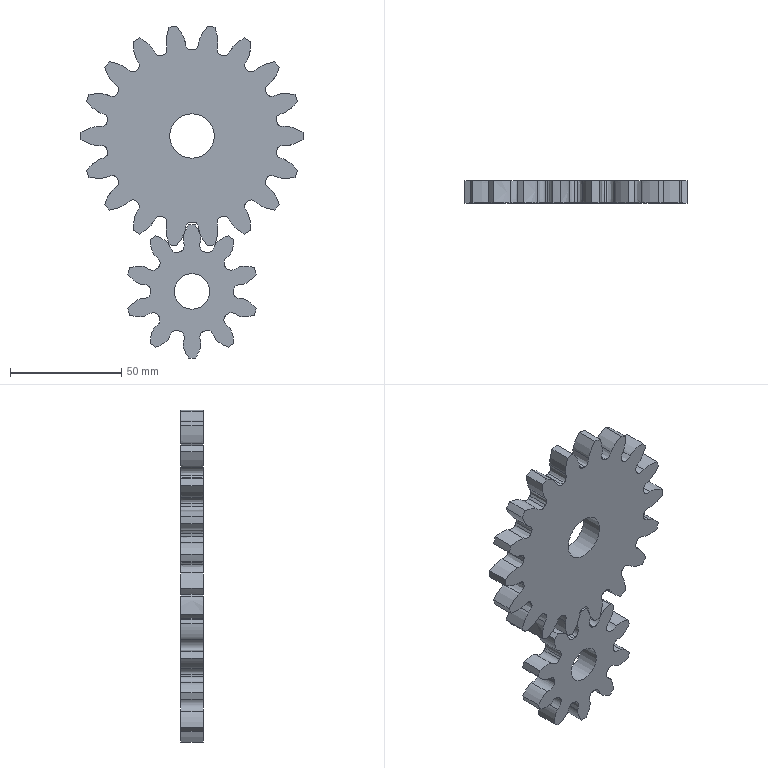Component | NX | SPUR_GEAR_SET | 2 solids | 174 faces | volume 75930 mm3 | other 90 | spline 50 | cylinder 30 | plane 4 | commonest cylinder face diameters 77.5 x18 37.46 x10 20 x1 16 x1